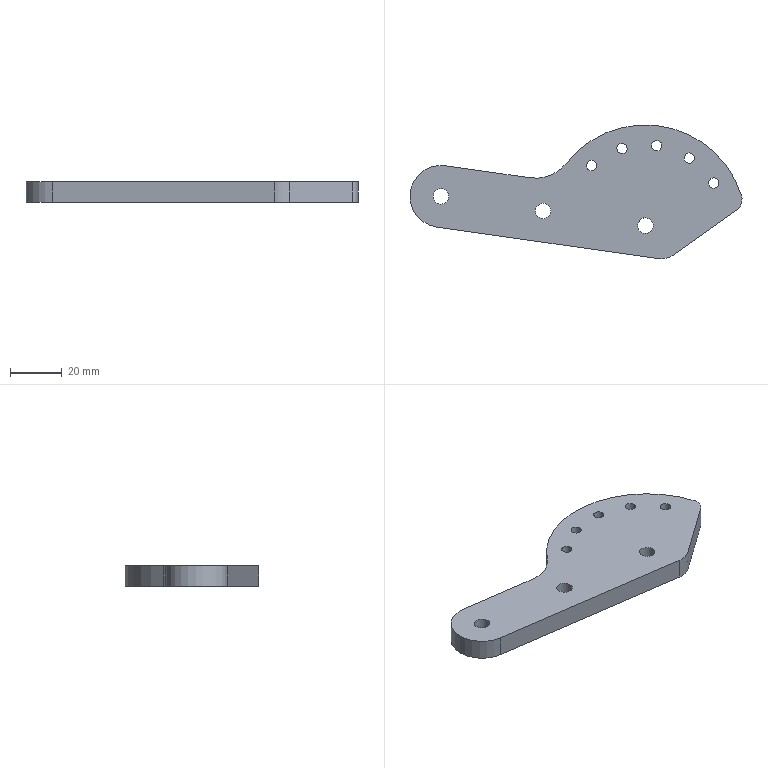Component | NX | 3 | 1 solid | 18 faces | volume 32162 mm3 | cylinder 13 | plane 5 | commonest cylinder face diameters 4 x5 6 x3 24 x1 16 x1 10 x1 78 x1 30 x1